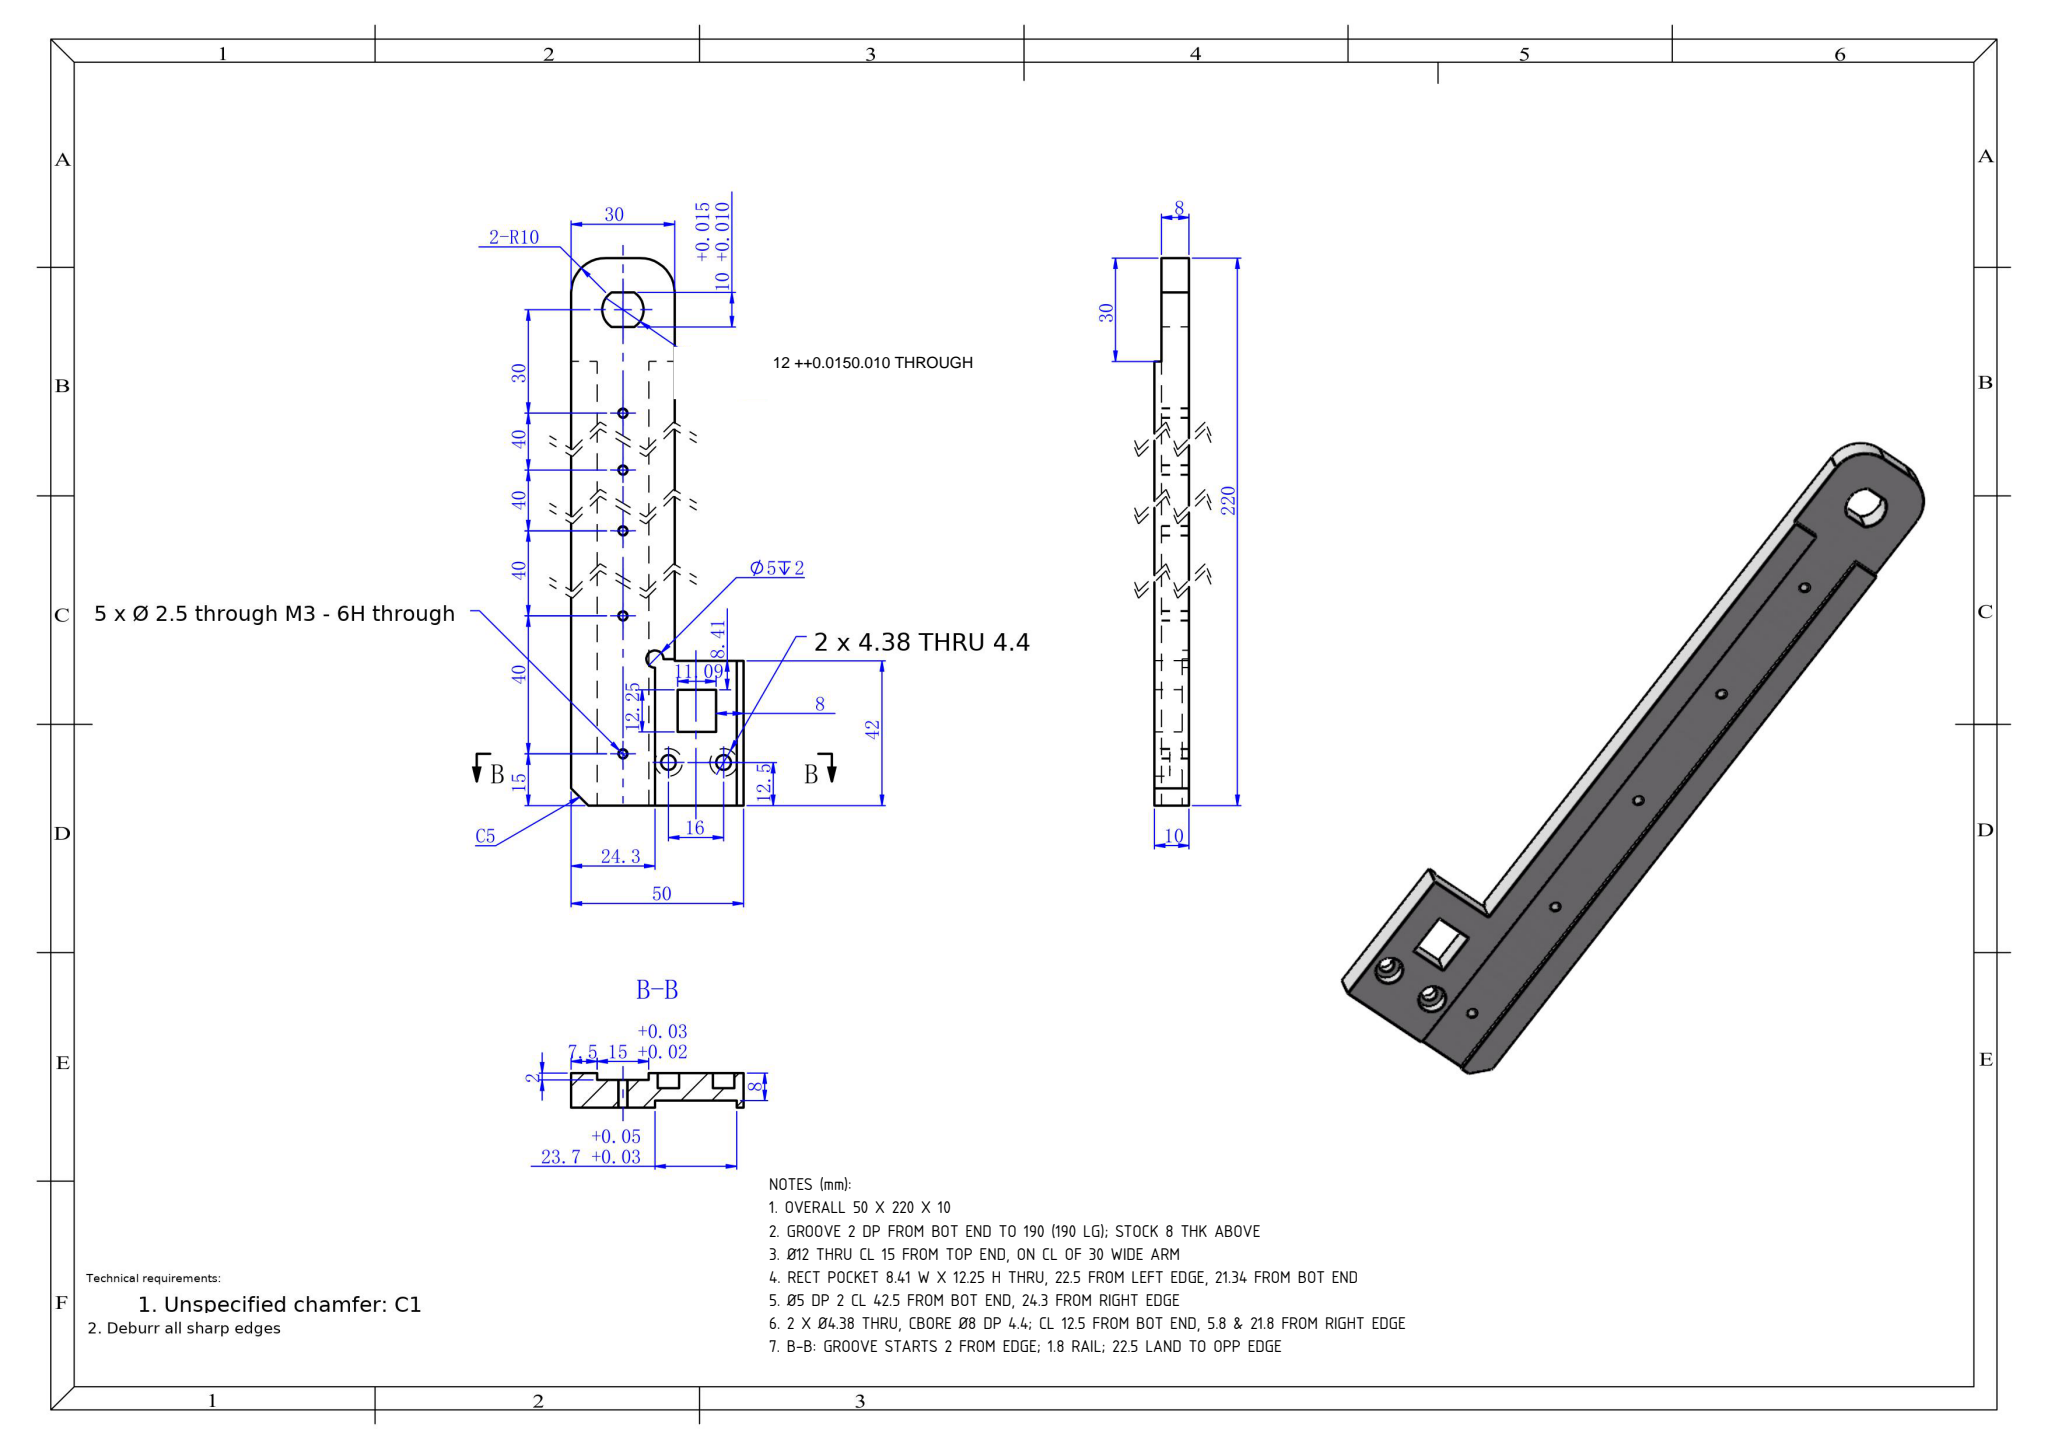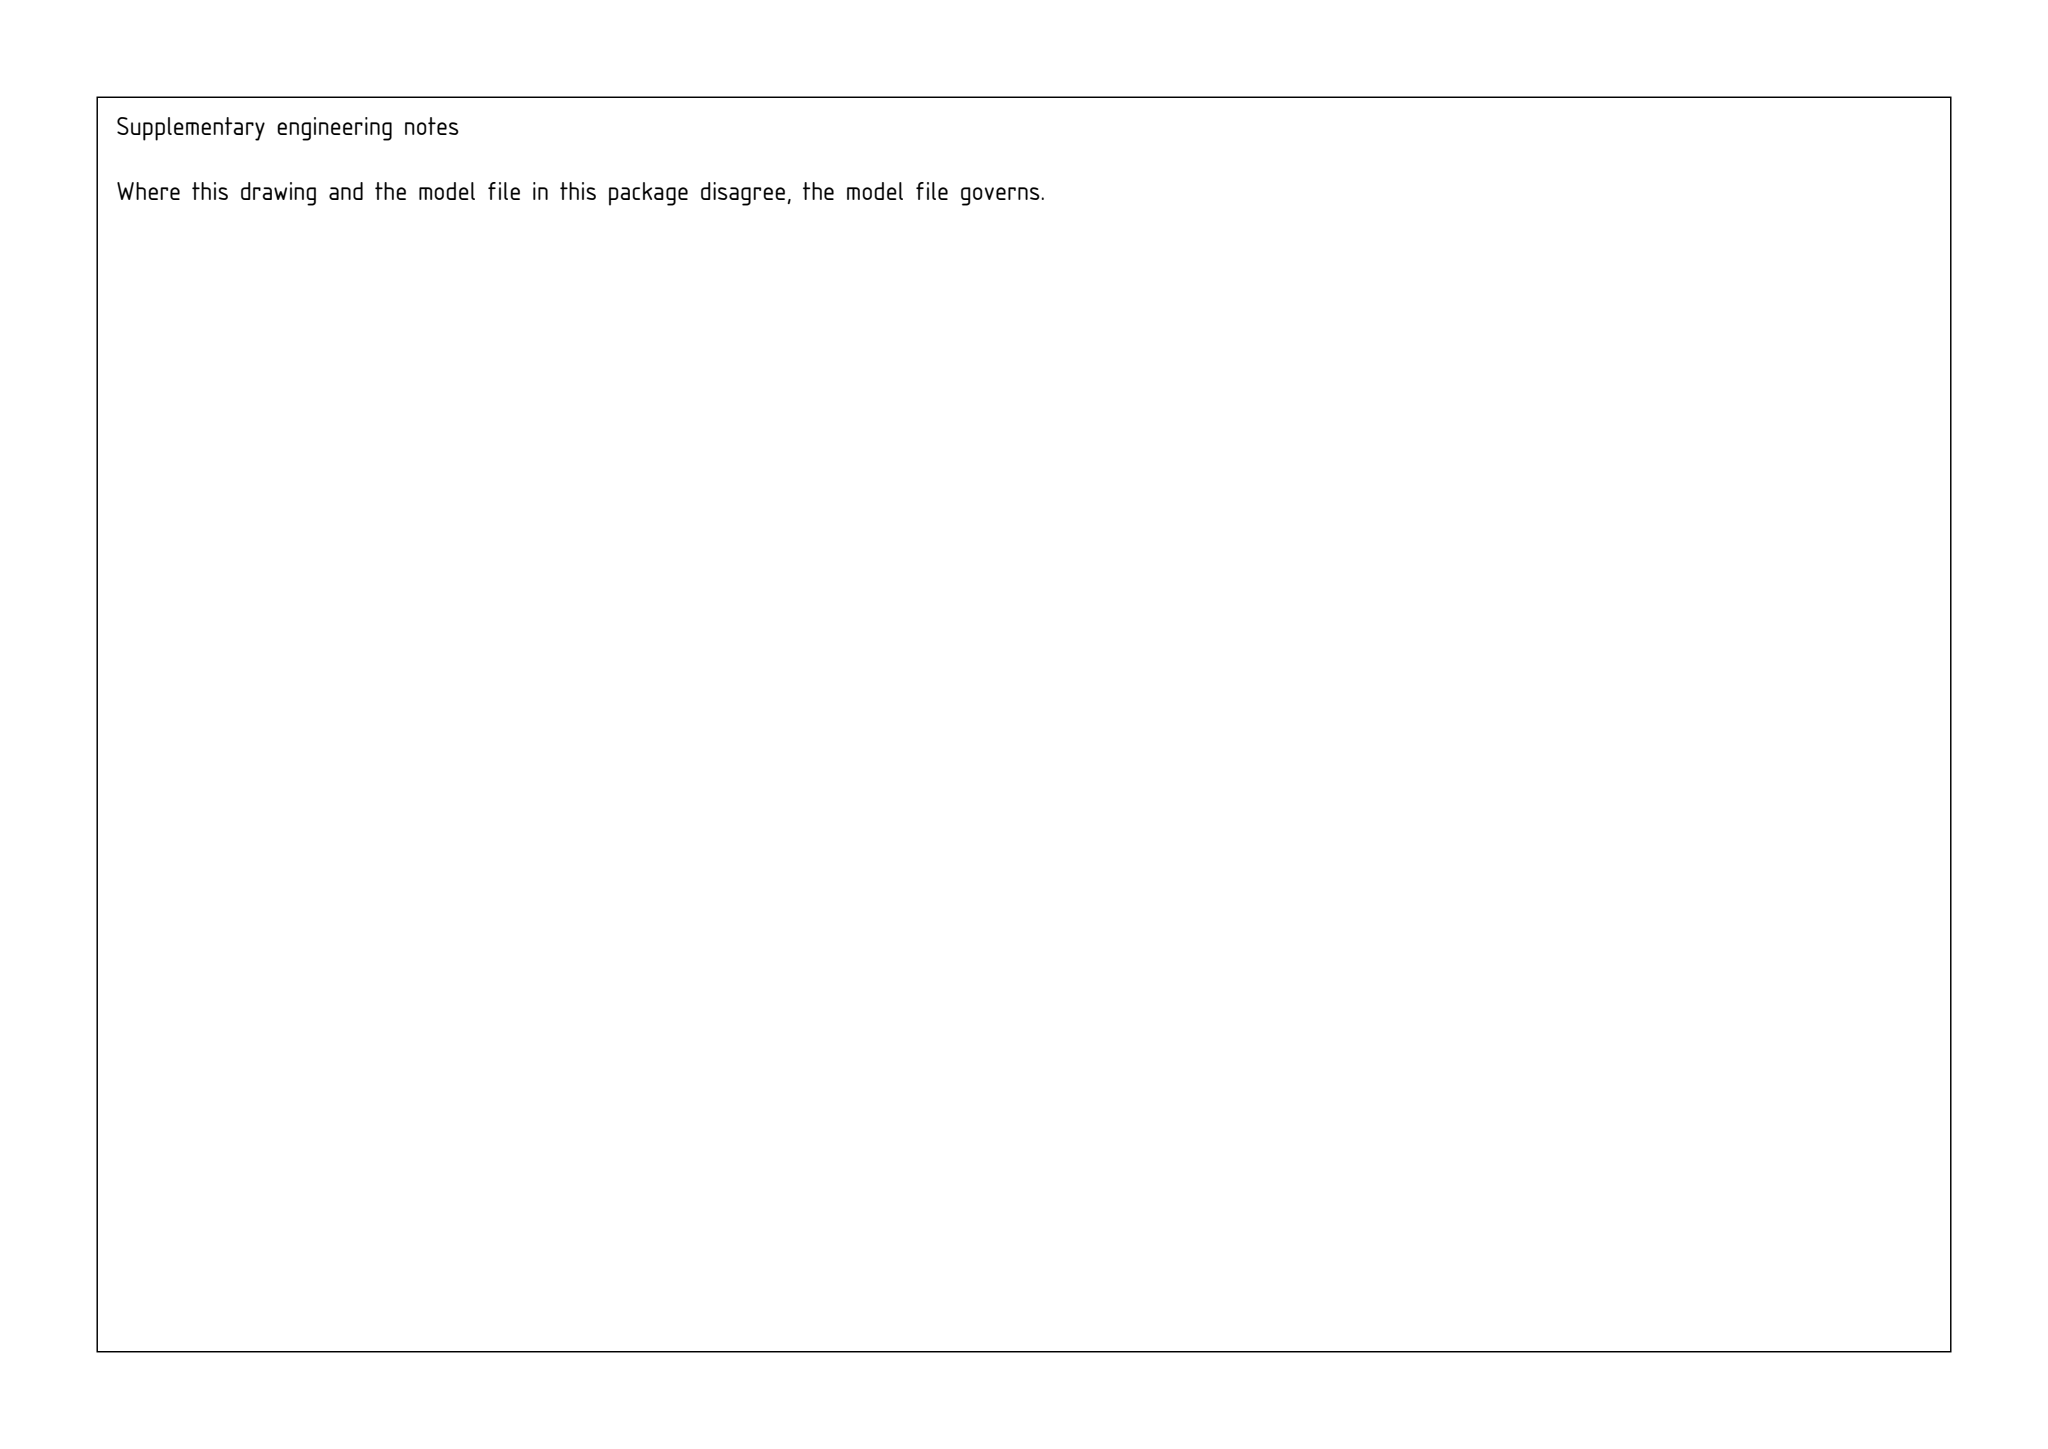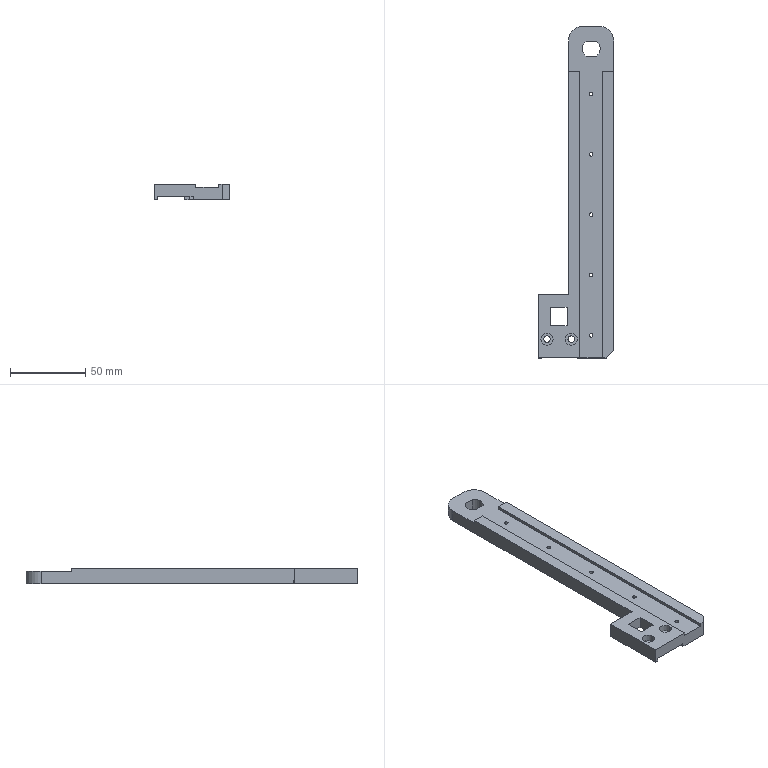Part | SolidWorks | mm | 1 solid | 52 faces | box 50 x 220 x 10 mm | volume 61743 mm3 | plane 28 | cylinder 24 | commonest cylinder face diameters 2.5 x10 8 x4 4.3 x4 12 x3 20 x2 5 x1
Drawing notes:
OVERALL 50 X 220 X 10 | from the solid: bbox_xyz 50 x 220 x 10
GROOVE 2 DP FROM BOT END TO 190 (190 LG); STOCK 8 THK ABOVE | from the solid: Z plane 8.0 (10-8=2 dp) bounded by Y planes 0.0 and 190.0
Ø12 THRU CL 15 FROM TOP END, ON CL OF 30 WIDE ARM | from the solid: Ø12 axis z at (35,205); 220-205=15 from top end; arm x20-50, CL x=35
RECT POCKET 8.41 W X 12.25 H THRU, 22.5 FROM LEFT EDGE, 21.34 FROM BOT END | from the solid: X planes 19.09/27.5 = 8.41 W; Y planes 21.34/33.59 = 12.25 H; no Z floor -> THRU; 50-27.5=22.5
Ø5 DP 2 CL 42.5 FROM BOT END, 24.3 FROM RIGHT EDGE | from the solid: cyl Ø5.0 axis z at [25.7,42.5], length 2.0; 50-25.7=24.3
2 X Ø4.38 THRU, CBORE Ø8 DP 4.4; CL 12.5 FROM BOT END, 5.8 & 21.8 FROM RIGHT EDGE | from the solid: Ø4.3 & Ø8 c'bore axes at (5.8,12.5) and (21.8,12.5), 16 apart; cbore length 4.4
B-B: GROOVE STARTS 2 FROM EDGE; 1.8 RAIL; 22.5 LAND TO OPP EDGE | from the solid: x-planes 0/2.0/25.7/27.5/50.0: 2 land, 23.7 groove (2>25.7), 1.8 rail (25.7>27.5), 22.5 land (27.5>50)